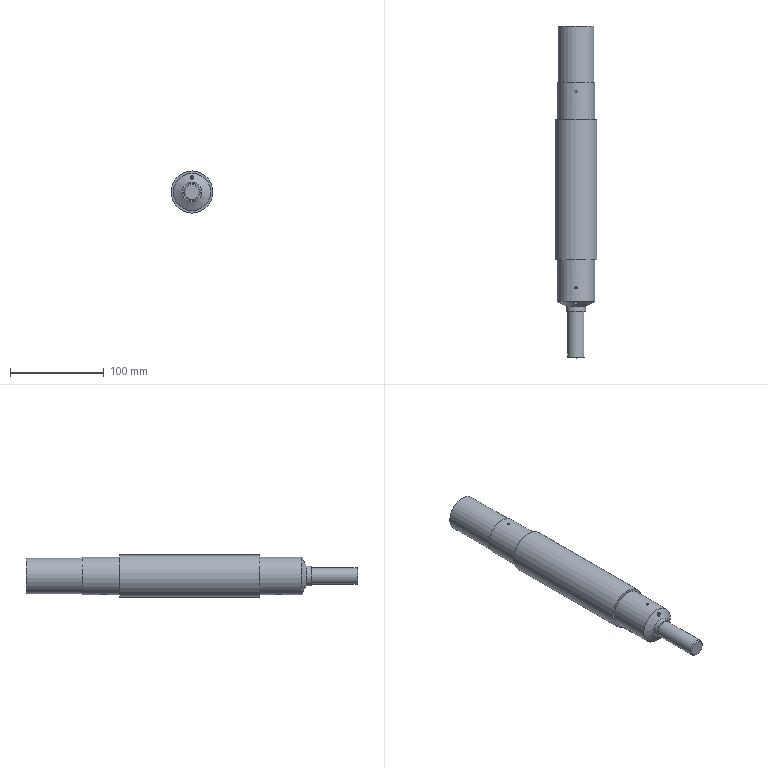Component | NX | 9_MANDREL | 1 solid | 31 faces | volume 413172 mm3 | cylinder 16 | cone 8 | plane 7 | commonest cylinder face diameters 2.5 x4 8 x3 40 x2 4.2 x2 38 x1 45 x1 21 x1 18 x1